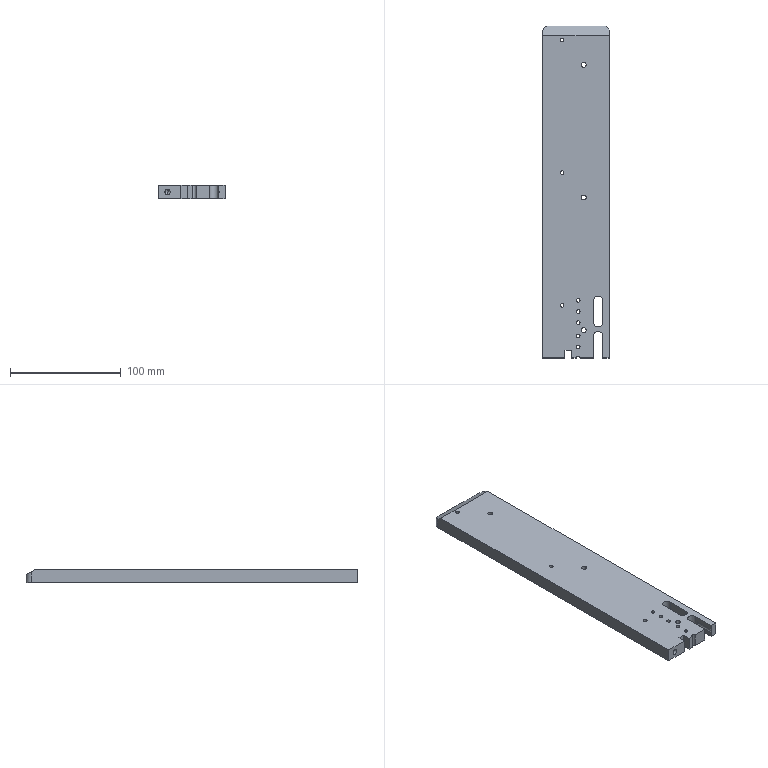Component | SolidWorks | 04-1111-1 | 1 solid | 66 faces | box 60 x 300 x 12 mm | volume 201035 mm3 | cylinder 39 | plane 24 | cone 3 | commonest cylinder face diameters 3.3 x17 8 x9 4.5 x6 5 x3 10 x2 4 x2
build123d program:
from build123d import *

# Parameters (mm, degrees)
SKETCH1_W                                       = 60
SKETCH1_H                                       = 12
BOSS_EXTRUDE1_DEPTH                             = 300
SKETCH2_W                                       = 20
SKETCH2_H                                       = 50
CUT_EXTRUDE1_DEPTH                              = 6
CUT_EXTRUDE2_DEPTH                              = 302.735
CHAMFER1_SIZE                                   = 5
CHAMFER1_SIZE2                                  = 8.66
FILLET1_R                                       = 5
SKETCH6_R                                       = 2
CUT_EXTRUDE3_DEPTH                              = 6
M6_TAPPED_HOLE1_D                               = 5
M6_TAPPED_HOLE1_DEPTH                           = 17
M6_TAPPED_HOLE1_TIP                             = 1.502
SKETCH9_W                                       = 6
SKETCH9_H                                       = 14
CUT_EXTRUDE4_DEPTH                              = 302.735
M4_HEX_SOCKET_HEAD_CAP_SCREW_CBORE1_D           = 4.5
M4_HEX_SOCKET_HEAD_CAP_SCREW_CBORE1_CBORE_D     = 8
M4_HEX_SOCKET_HEAD_CAP_SCREW_CBORE1_CBORE_DEPTH = 4.4
M4_TAPPED_HOLE1_D                               = 3.3
LPATTERN1_COUNT                                 = 2
LPATTERN1_PITCH                                 = 32
M4_TAPPED_HOLE2_D                               = 3.3


with BuildPart() as part:
    # Sketch1 → Boss-Extrude1 (new body)
    with BuildSketch(Plane(origin=(0, 0, 0), x_dir=(1, 0, 0), z_dir=(0, 1, 0))):
        Rectangle(SKETCH1_W, SKETCH1_H)
    extrude(amount=BOSS_EXTRUDE1_DEPTH)

    # Sketch2 → Cut-Extrude1 (cut)
    with BuildSketch(Plane.XY.offset(-6)):
        with Locations((-20, 190)):
            Rectangle(SKETCH2_W, SKETCH2_H)
    extrude(amount=CUT_EXTRUDE1_DEPTH, mode=Mode.SUBTRACT)

    # Sketch3 → Cut-Extrude2 (cut, through all)
    with BuildSketch(Plane(origin=(0, 0, -6), x_dir=(-1, 0, 0), z_dir=(0, 0, -1))):
        with BuildLine():
            Line((24, 300), (24, 280))
            ThreePointArc((24, 280), (20, 276), (16, 280))
            Line((16, 280), (16, 300))
            ThreePointArc((16, 300), (20, 304), (24, 300))
        make_face()
    cut_extrude2 = extrude(amount=-CUT_EXTRUDE2_DEPTH, mode=Mode.SUBTRACT)

    # Chamfer1
    chamfer1_edges = [part.edges().sort_by_distance(p)[0] for p in [
        (0, 0, 6),
    ]]
    chamfer1_side = [part.faces().sort_by_distance(p)[0] for p in [
        (0, 0, 0),
    ]]
    chamfer(chamfer1_edges, length=CHAMFER1_SIZE, length2=CHAMFER1_SIZE2, reference=chamfer1_side[0])

    # Fillet1
    fillet1_edges = [part.edges().sort_by_distance(p)[0] for p in [
        (30, 0, -2.5),
        (-30, 0, -2.5),
    ]]
    fillet(fillet1_edges, radius=FILLET1_R)

    # Sketch6 → Cut-Extrude3 (cut)
    with BuildSketch(Plane(origin=(0, 0, -6), x_dir=(-1, 0, 0), z_dir=(0, 0, -1))):
        with Locations((10, 167)):
            Circle(SKETCH6_R)
        with Locations((10, 213)):
            Circle(SKETCH6_R)
    extrude(amount=-CUT_EXTRUDE3_DEPTH, mode=Mode.SUBTRACT)

    # M6 Tapped Hole1
    with Locations(Plane(origin=(0, 300, 0), x_dir=(1, 0, 0), z_dir=(0, 1, 0))):
        with Locations((-22, 0), (22, 0)):
            Hole(M6_TAPPED_HOLE1_D / 2, depth=M6_TAPPED_HOLE1_DEPTH)
            with Locations((0, 0, -(M6_TAPPED_HOLE1_DEPTH + M6_TAPPED_HOLE1_TIP / 2))):  # 118° drill point
                Cone(0, M6_TAPPED_HOLE1_D / 2, M6_TAPPED_HOLE1_TIP, mode=Mode.SUBTRACT)

    # Sketch9 → Cut-Extrude4 (cut, through all)
    with BuildSketch(Plane(origin=(0, 0, -6), x_dir=(-1, 0, 0), z_dir=(0, 0, -1))):
        with Locations((-7, 300)):
            Rectangle(SKETCH9_W, SKETCH9_H)
    extrude(amount=-CUT_EXTRUDE4_DEPTH, mode=Mode.SUBTRACT)

    # M4 Hex Socket Head Cap Screw CBORE1 (through all)
    with Locations(Plane(origin=(0, 0, -6), x_dir=(-1, 0, 0), z_dir=(0, 0, -1))):
        with Locations((7, 35), (7, 155), (7, 275)):
            CounterBoreHole(M4_HEX_SOCKET_HEAD_CAP_SCREW_CBORE1_D / 2, M4_HEX_SOCKET_HEAD_CAP_SCREW_CBORE1_CBORE_D / 2, M4_HEX_SOCKET_HEAD_CAP_SCREW_CBORE1_CBORE_DEPTH)

    # M4 Tapped Hole1 (through all)
    with Locations(Plane(origin=(0, 0, -6), x_dir=(-1, 0, 0), z_dir=(0, 0, -1))):
        with Locations((2, 280), (2, 290), (2, 300)):
            m4_tapped_hole1 = Hole(M4_TAPPED_HOLE1_D / 2)

    # LPattern1: Cut-Extrude2, M4 Tapped Hole1 ×2
    with Locations(*[(0, -i * LPATTERN1_PITCH, 0) for i in range(1, LPATTERN1_COUNT)]):
        add(cut_extrude2, mode=Mode.SUBTRACT)
        add(m4_tapped_hole1, mode=Mode.SUBTRACT)

    # M4 Tapped Hole2 (through all)
    with Locations(Plane.XY.offset(6)):
        with Locations((12.5, 12.5), (12.5, 132.5), (12.5, 252.5)):
            Hole(M4_TAPPED_HOLE2_D / 2)


solid = part.part

# Placed as in the assembly
solid = solid.moved(Location((-135.072, 706.224, 1276.056), (0, 0, 180)))